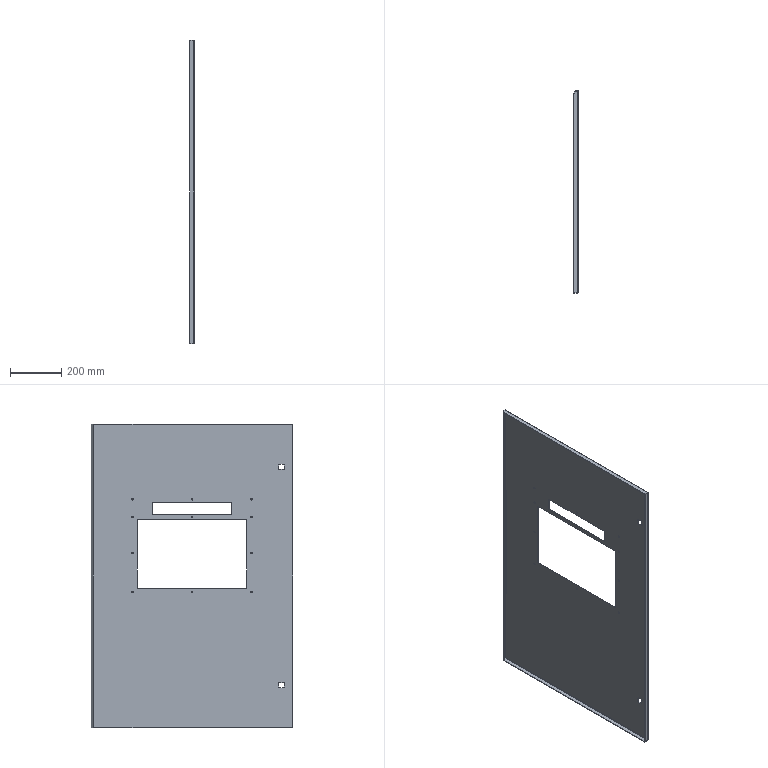Component | SolidWorks | FrontMiddleLowerDoor-1_FrontMiddleLowerDoor-1 | 1 solid | 101 faces | volume 1742700 mm3 | plane 57 | cylinder 40 | spline 4 | commonest cylinder face diameters 6 x35 2 x5